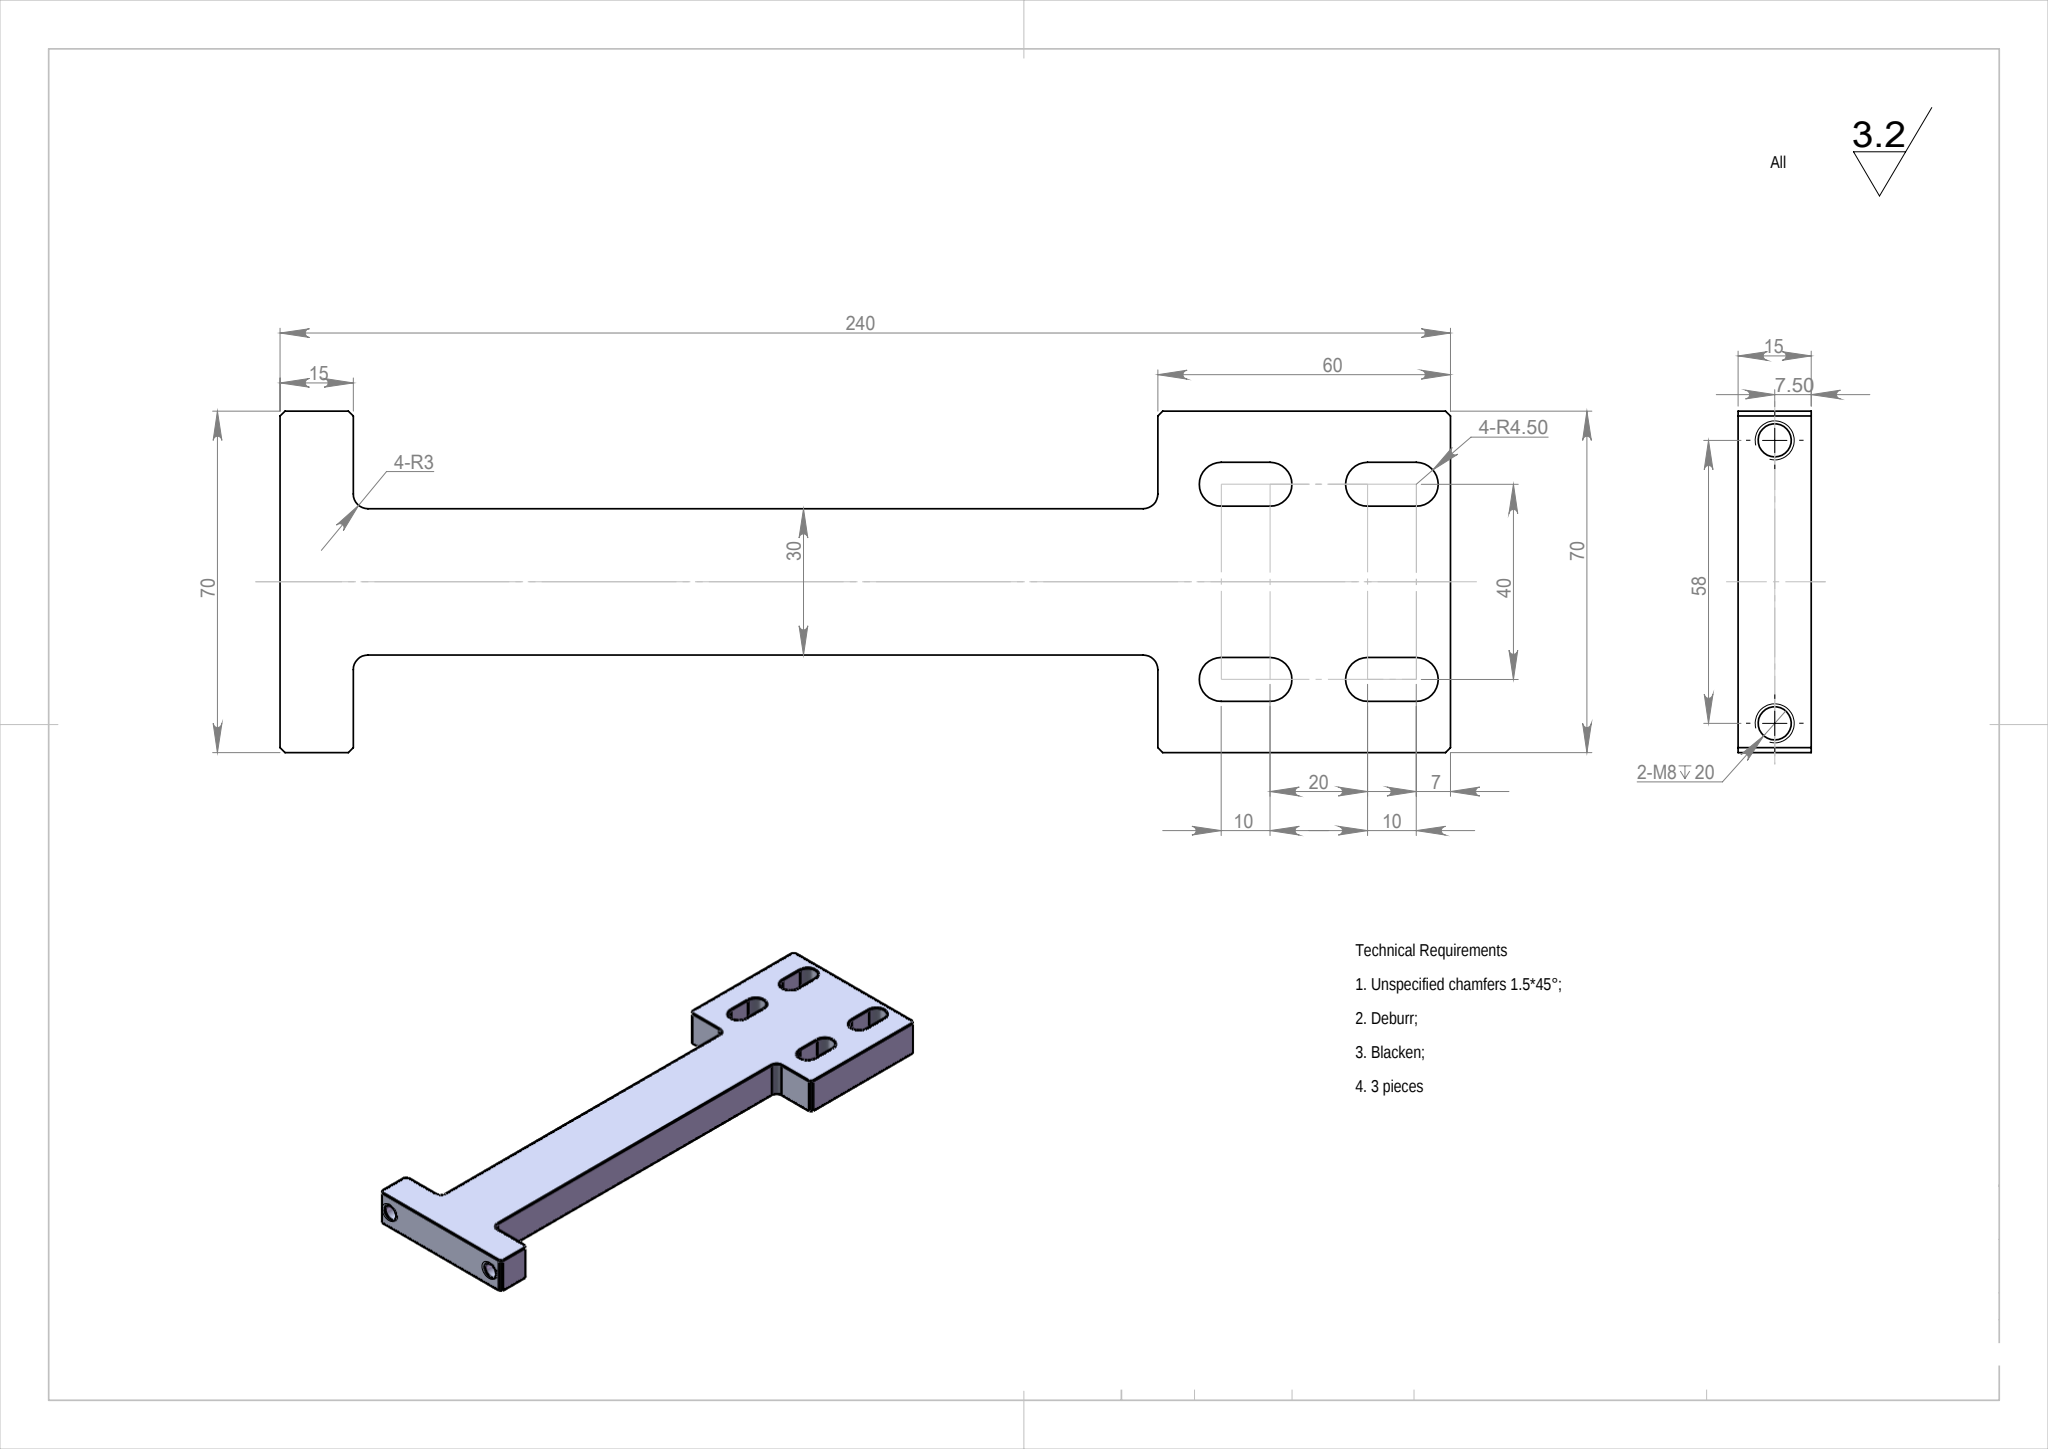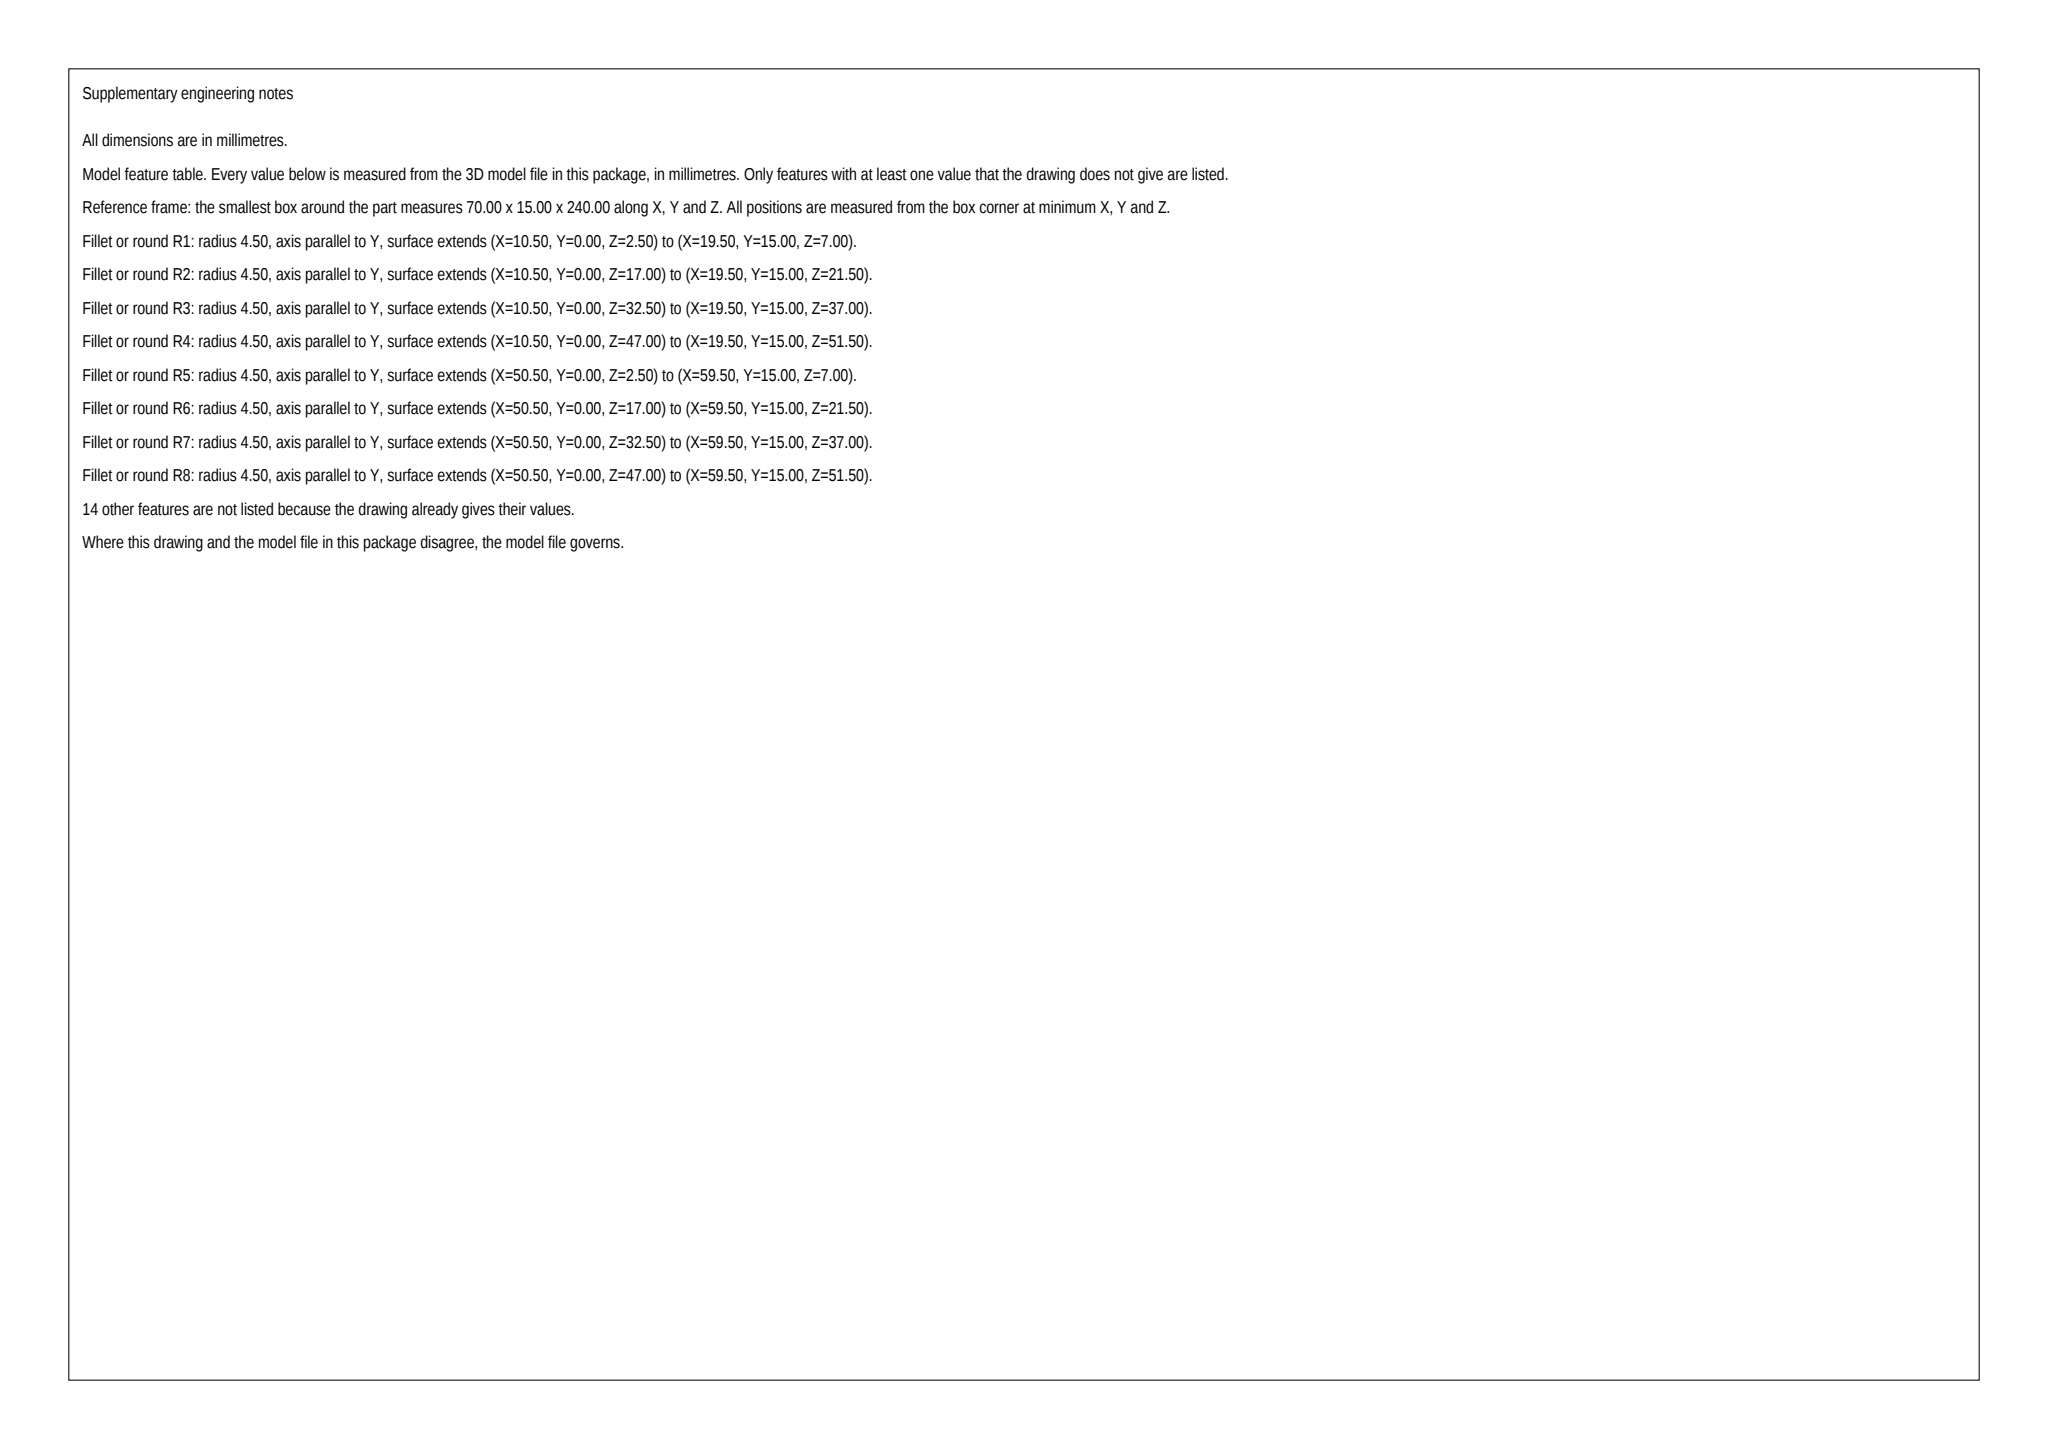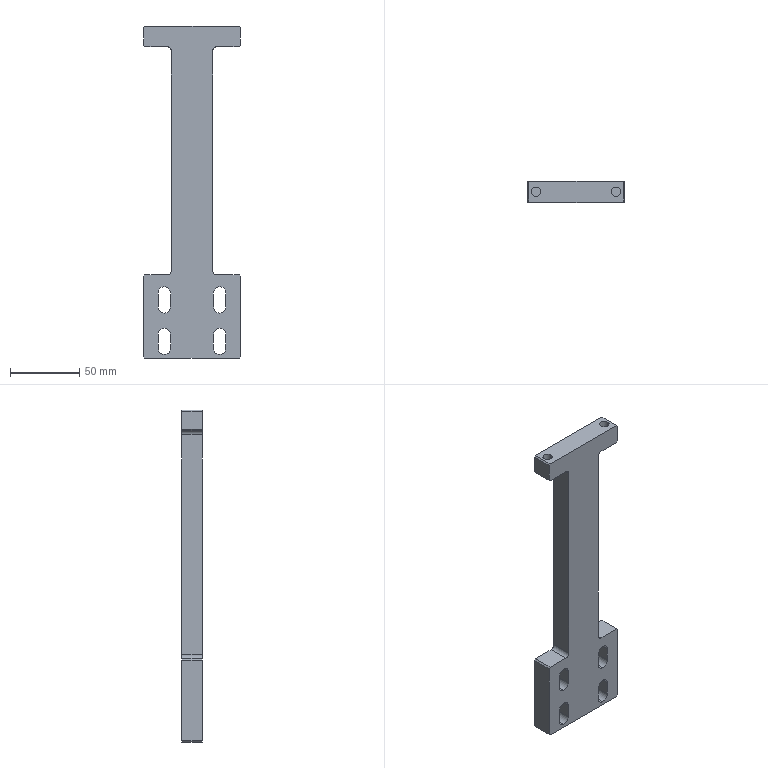Part | SolidWorks | mm | 1 solid | 50 faces | box 70 x 15 x 240 mm | volume 142749 mm3 | plane 30 | cylinder 20 | commonest cylinder face diameters 9 x12 6.8 x4 6 x4
build123d program:
from build123d import *

# Parameters (mm, degrees)
SKETCH1_W              = 70
SKETCH1_H              = 15
BOSS_EXTRUDE1_DEPTH    = 120
SKETCH2_W              = 20
SKETCH2_H              = 165
CUT_EXTRUDE1_DEPTH     = 126.897
FILLET1_R              = 3
CHAMFER1_SIZE          = 1
M8_TAPPED_HOLE1_D      = 6.8
M8_TAPPED_HOLE1_DEPTH  = 22.25
M8_TAPPED_HOLE1_TIP    = 2.043
CUT_EXTRUDE2_DEPTH     = 126.897
LPATTERN1_COUNT        = 2
LPATTERN1_PITCH        = 30
LPATTERN1_COPY_1_DEPTH = 126.897


with BuildPart() as part:
    # Sketch1 → Boss-Extrude1 (new, symmetric)
    with BuildSketch(Plane.XY):
        Rectangle(SKETCH1_W, SKETCH1_H)
    extrude(amount=BOSS_EXTRUDE1_DEPTH, both=True)

    # Sketch2 → Cut-Extrude1 (cut, through all)
    with BuildSketch(Plane(origin=(0, 7.5, 0), x_dir=(1, 0, 0), z_dir=(0, 1, 0))):
        with Locations((-25, -22.5)):
            Rectangle(SKETCH2_W, SKETCH2_H)
    cut_extrude1 = extrude(amount=-CUT_EXTRUDE1_DEPTH, mode=Mode.SUBTRACT)

    # Mirror1: Cut-Extrude1 across plane
    add(cut_extrude1.mirror(Plane(origin=(0, 0, 0), x_dir=(0, 0, 1), z_dir=(1, 0, 0))), mode=Mode.SUBTRACT)

    # Fillet1
    fillet1_edges = [part.edges().sort_by_distance(p)[0] for p in [
        (-15, 0, -60),
        (-15, 0, 105),
        (15, 0, 105),
        (15, 0, -60),
    ]]
    fillet(fillet1_edges, radius=FILLET1_R)

    # Chamfer1
    chamfer1_edges = [part.edges().sort_by_distance(p)[0] for p in [
        (-35, 0, 120),
        (-35, 0, 105),
        (-35, 0, -60),
        (35, 0, -60),
        (35, 0, 105),
        (35, 0, 120),
        (-35, 0, -120),
        (35, 0, -120),
    ]]
    chamfer(chamfer1_edges, length=CHAMFER1_SIZE)

    # M8 Tapped Hole1
    with Locations(Plane.XY.offset(120)):
        with Locations((-29, 0), (29, 0)):
            Hole(M8_TAPPED_HOLE1_D / 2, depth=M8_TAPPED_HOLE1_DEPTH)
            with Locations((0, 0, -(M8_TAPPED_HOLE1_DEPTH + M8_TAPPED_HOLE1_TIP / 2))):  # 118° drill point
                Cone(0, M8_TAPPED_HOLE1_D / 2, M8_TAPPED_HOLE1_TIP, mode=Mode.SUBTRACT)

    # Sketch5 → Cut-Extrude2 (cut, through all)
    with BuildSketch(Plane.XZ.offset(7.5)):
        with BuildLine():
            Line((-15.5, -103), (-15.5, -113))
            ThreePointArc((-15.5, -113), (-20, -117.5), (-24.5, -113))
            Line((-24.5, -113), (-24.5, -103))
            ThreePointArc((-24.5, -103), (-20, -98.5), (-15.5, -103))
        make_face()
    cut_extrude2 = extrude(amount=-CUT_EXTRUDE2_DEPTH, mode=Mode.SUBTRACT)

    # Mirror2: Cut-Extrude2 across plane
    add(cut_extrude2.mirror(Plane(origin=(0, 0, 0), x_dir=(0, 0, 1), z_dir=(1, 0, 0))), mode=Mode.SUBTRACT)

    # LPattern1: Cut-Extrude2 ×2
    with Locations(*[(0, 0, i * LPATTERN1_PITCH) for i in range(1, LPATTERN1_COUNT)]):
        add(cut_extrude2, mode=Mode.SUBTRACT)

    # LPattern1 copy 1 sketch → LPattern1 copy 1 (cut, through all)
    with BuildSketch(Plane(origin=(0, -7.5, 30), x_dir=(-1, 0, 0), z_dir=(0, -1, 0))):
        with BuildLine():
            Line((-15.5, 103), (-15.5, 113))
            ThreePointArc((-15.5, 113), (-20, 117.5), (-24.5, 113))
            Line((-24.5, 113), (-24.5, 103))
            ThreePointArc((-24.5, 103), (-20, 98.5), (-15.5, 103))
        make_face()
    extrude(amount=-LPATTERN1_COPY_1_DEPTH, mode=Mode.SUBTRACT)


solid = part.part